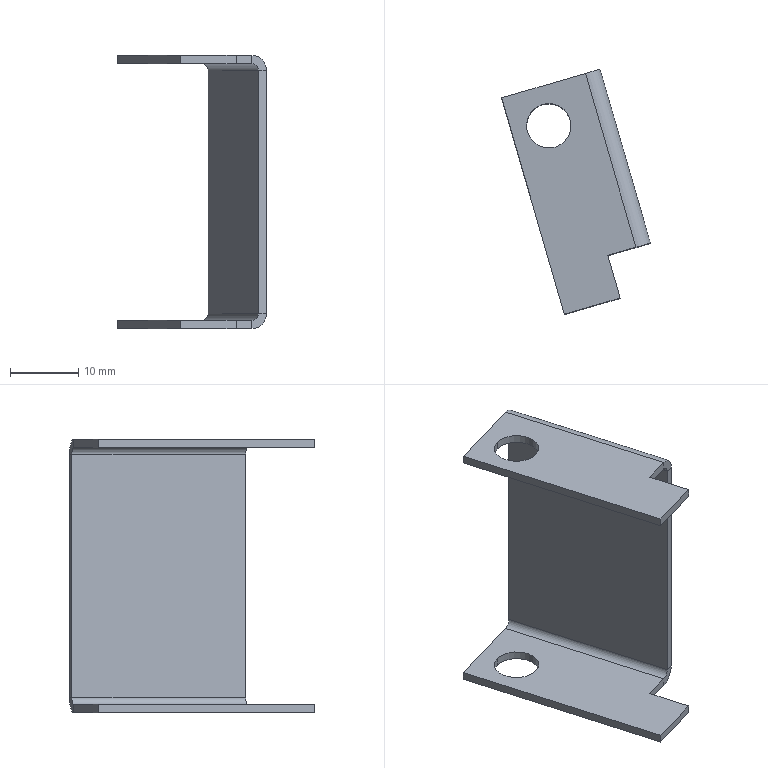Component | SolidWorks | LeftDoorAssembly-1_Bracket-1 | 1 solid | 30 faces | box 21.79 x 35.87 x 40 mm | volume 2159 mm3 | plane 22 | cylinder 8 | commonest cylinder face diameters 6.5 x4 4.4 x2 2 x2
STEP:
#1=CARTESIAN_POINT('',(10.397,8.439,58.906));
#2=VERTEX_POINT('',#1);
#3=CARTESIAN_POINT('',(10.325,8.685,58.906));
#4=VERTEX_POINT('',#3);
#5=CARTESIAN_POINT('',(10.361,8.562,58.906));
#6=DIRECTION('',(-0.,0.,1.));
#7=DIRECTION('',(-0.2786,0.9604,0.));
#8=AXIS2_PLACEMENT_3D('',#5,#6,#7);
#9=CIRCLE('',#8,0.128);
#10=EDGE_CURVE('',#2,#4,#9,.T.);
#11=ORIENTED_EDGE('',*,*,#10,.F.);
#12=CARTESIAN_POINT('',(10.397,8.439,58.953));
#13=VERTEX_POINT('',#12);
#14=CARTESIAN_POINT('',(10.397,8.439,58.906));
#15=DIRECTION('',(-0.,0.,1.));
#16=VECTOR('',#15,39.37);
#17=LINE('',#14,#16);
#18=EDGE_CURVE('',#2,#13,#17,.T.);
#19=ORIENTED_EDGE('',*,*,#18,.T.);
#20=CARTESIAN_POINT('',(10.325,8.685,58.953));
#21=VERTEX_POINT('',#20);
#22=CARTESIAN_POINT('',(10.361,8.562,58.953));
#23=DIRECTION('',(-0.,0.,1.));
#24=DIRECTION('',(-0.2786,0.9604,0.));
#25=AXIS2_PLACEMENT_3D('',#22,#23,#24);
#26=CIRCLE('',#25,0.128);
#27=EDGE_CURVE('',#13,#21,#26,.T.);
#28=ORIENTED_EDGE('',*,*,#27,.T.);
#29=CARTESIAN_POINT('',(10.325,8.685,58.906));
#30=DIRECTION('',(-0.,0.,1.));
#31=VECTOR('',#30,39.37);
#32=LINE('',#29,#31);
#33=EDGE_CURVE('',#4,#21,#32,.T.);
#34=ORIENTED_EDGE('',*,*,#33,.F.);
#35=EDGE_LOOP('',(#11,#19,#28,#34));
#36=FACE_OUTER_BOUND('',#35,.T.);
#37=CARTESIAN_POINT('',(10.361,8.562,58.906));
#38=DIRECTION('',(-0.,0.,1.));
#39=DIRECTION('',(-0.2786,0.9604,0.));
#40=AXIS2_PLACEMENT_3D('',#37,#38,#39);
#41=CYLINDRICAL_SURFACE('',#40,0.128);
#42=ADVANCED_FACE('',(#36),#41,.F.);
#43=CARTESIAN_POINT('',(10.397,8.439,60.433));
#44=VERTEX_POINT('',#43);
#45=CARTESIAN_POINT('',(10.325,8.685,60.433));
#46=VERTEX_POINT('',#45);
#47=CARTESIAN_POINT('',(10.361,8.562,60.433));
#48=DIRECTION('',(-0.,0.,1.));
#49=DIRECTION('',(-0.2786,0.9604,0.));
#50=AXIS2_PLACEMENT_3D('',#47,#48,#49);
#51=CIRCLE('',#50,0.128);
#52=EDGE_CURVE('',#44,#46,#51,.T.);
#53=ORIENTED_EDGE('',*,*,#52,.F.);
#54=CARTESIAN_POINT('',(10.397,8.439,60.48));
#55=VERTEX_POINT('',#54);
#56=CARTESIAN_POINT('',(10.397,8.439,60.48));
#57=DIRECTION('',(-0.,0.,1.));
#58=VECTOR('',#57,39.37);
#59=LINE('',#56,#58);
#60=EDGE_CURVE('',#44,#55,#59,.T.);
#61=ORIENTED_EDGE('',*,*,#60,.T.);
#62=CARTESIAN_POINT('',(10.325,8.685,60.48));
#63=VERTEX_POINT('',#62);
#64=CARTESIAN_POINT('',(10.361,8.562,60.48));
#65=DIRECTION('',(-0.,0.,1.));
#66=DIRECTION('',(-0.2786,0.9604,0.));
#67=AXIS2_PLACEMENT_3D('',#64,#65,#66);
#68=CIRCLE('',#67,0.128);
#69=EDGE_CURVE('',#55,#63,#68,.T.);
#70=ORIENTED_EDGE('',*,*,#69,.T.);
#71=CARTESIAN_POINT('',(10.325,8.685,60.48));
#72=DIRECTION('',(-0.,0.,1.));
#73=VECTOR('',#72,39.37);
#74=LINE('',#71,#73);
#75=EDGE_CURVE('',#46,#63,#74,.T.);
#76=ORIENTED_EDGE('',*,*,#75,.F.);
#77=EDGE_LOOP('',(#53,#61,#70,#76));
#78=FACE_OUTER_BOUND('',#77,.T.);
#79=CARTESIAN_POINT('',(10.361,8.562,60.48));
#80=DIRECTION('',(-0.,0.,1.));
#81=DIRECTION('',(-0.2786,0.9604,0.));
#82=AXIS2_PLACEMENT_3D('',#79,#80,#81);
#83=CYLINDRICAL_SURFACE('',#82,0.128);
#84=ADVANCED_FACE('',(#78),#83,.F.);
#85=CARTESIAN_POINT('',(10.361,8.562,58.906));
#86=DIRECTION('',(-0.,0.,1.));
#87=DIRECTION('',(-0.2786,0.9604,0.));
#88=AXIS2_PLACEMENT_3D('',#85,#86,#87);
#89=CIRCLE('',#88,0.128);
#90=EDGE_CURVE('',#4,#2,#89,.T.);
#91=ORIENTED_EDGE('',*,*,#90,.T.);
#92=ORIENTED_EDGE('',*,*,#10,.T.);
#93=EDGE_LOOP('',(#91,#92));
#94=FACE_BOUND('',#93,.T.);
#95=CARTESIAN_POINT('',(10.863,7.862,58.906));
#96=VERTEX_POINT('',#95);
#97=CARTESIAN_POINT('',(10.573,8.864,58.906));
#98=VERTEX_POINT('',#97);
#99=CARTESIAN_POINT('',(10.935,7.616,58.906));
#100=DIRECTION('',(-0.2786,0.9604,-0.));
#101=VECTOR('',#100,39.37);
#102=LINE('',#99,#101);
#103=EDGE_CURVE('',#96,#98,#102,.T.);
#104=ORIENTED_EDGE('',*,*,#103,.F.);
#105=CARTESIAN_POINT('',(10.701,7.815,58.906));
#106=VERTEX_POINT('',#105);
#107=CARTESIAN_POINT('',(10.901,7.873,58.906));
#108=DIRECTION('',(0.9604,0.2786,0.));
#109=VECTOR('',#108,39.37);
#110=LINE('',#107,#109);
#111=EDGE_CURVE('',#106,#96,#110,.T.);
#112=ORIENTED_EDGE('',*,*,#111,.F.);
#113=CARTESIAN_POINT('',(10.772,7.569,58.906));
#114=VERTEX_POINT('',#113);
#115=CARTESIAN_POINT('',(10.772,7.569,58.906));
#116=DIRECTION('',(-0.2786,0.9604,-0.));
#117=VECTOR('',#116,39.37);
#118=LINE('',#115,#117);
#119=EDGE_CURVE('',#114,#106,#118,.T.);
#120=ORIENTED_EDGE('',*,*,#119,.F.);
#121=CARTESIAN_POINT('',(10.451,7.476,58.906));
#122=VERTEX_POINT('',#121);
#123=CARTESIAN_POINT('',(10.973,7.627,58.906));
#124=DIRECTION('',(-0.9604,-0.2786,-0.));
#125=VECTOR('',#124,39.37);
#126=LINE('',#123,#125);
#127=EDGE_CURVE('',#114,#122,#126,.T.);
#128=ORIENTED_EDGE('',*,*,#127,.T.);
#129=CARTESIAN_POINT('',(10.089,8.723,58.906));
#130=VERTEX_POINT('',#129);
#131=CARTESIAN_POINT('',(10.451,7.476,58.906));
#132=DIRECTION('',(-0.2786,0.9604,-0.));
#133=VECTOR('',#132,39.37);
#134=LINE('',#131,#133);
#135=EDGE_CURVE('',#122,#130,#134,.T.);
#136=ORIENTED_EDGE('',*,*,#135,.T.);
#137=CARTESIAN_POINT('',(10.611,8.875,58.906));
#138=DIRECTION('',(-0.9604,-0.2786,-0.));
#139=VECTOR('',#138,39.37);
#140=LINE('',#137,#139);
#141=EDGE_CURVE('',#98,#130,#140,.T.);
#142=ORIENTED_EDGE('',*,*,#141,.F.);
#143=EDGE_LOOP('',(#104,#112,#120,#128,#136,#142));
#144=FACE_OUTER_BOUND('',#143,.T.);
#145=CARTESIAN_POINT('',(10.973,7.627,58.906));
#146=DIRECTION('',(0.,-0.,-1.));
#147=DIRECTION('',(0.2786,-0.9604,0.));
#148=AXIS2_PLACEMENT_3D('',#145,#146,#147);
#149=PLANE('',#148);
#150=ADVANCED_FACE('',(#94,#144),#149,.T.);
#151=CARTESIAN_POINT('',(10.361,8.562,58.953));
#152=DIRECTION('',(-0.,0.,1.));
#153=DIRECTION('',(-0.2786,0.9604,0.));
#154=AXIS2_PLACEMENT_3D('',#151,#152,#153);
#155=CIRCLE('',#154,0.128);
#156=EDGE_CURVE('',#21,#13,#155,.T.);
#157=ORIENTED_EDGE('',*,*,#156,.F.);
#158=ORIENTED_EDGE('',*,*,#27,.F.);
#159=EDGE_LOOP('',(#157,#158));
#160=FACE_BOUND('',#159,.T.);
#161=CARTESIAN_POINT('',(10.701,7.815,58.953));
#162=VERTEX_POINT('',#161);
#163=CARTESIAN_POINT('',(10.863,7.862,58.953));
#164=VERTEX_POINT('',#163);
#165=CARTESIAN_POINT('',(10.901,7.873,58.953));
#166=DIRECTION('',(0.9604,0.2786,0.));
#167=VECTOR('',#166,39.37);
#168=LINE('',#165,#167);
#169=EDGE_CURVE('',#162,#164,#168,.T.);
#170=ORIENTED_EDGE('',*,*,#169,.T.);
#171=CARTESIAN_POINT('',(10.573,8.864,58.953));
#172=VERTEX_POINT('',#171);
#173=CARTESIAN_POINT('',(10.935,7.616,58.953));
#174=DIRECTION('',(-0.2786,0.9604,-0.));
#175=VECTOR('',#174,39.37);
#176=LINE('',#173,#175);
#177=EDGE_CURVE('',#164,#172,#176,.T.);
#178=ORIENTED_EDGE('',*,*,#177,.T.);
#179=CARTESIAN_POINT('',(10.089,8.723,58.953));
#180=VERTEX_POINT('',#179);
#181=CARTESIAN_POINT('',(10.611,8.875,58.953));
#182=DIRECTION('',(-0.9604,-0.2786,-0.));
#183=VECTOR('',#182,39.37);
#184=LINE('',#181,#183);
#185=EDGE_CURVE('',#172,#180,#184,.T.);
#186=ORIENTED_EDGE('',*,*,#185,.T.);
#187=CARTESIAN_POINT('',(10.451,7.476,58.953));
#188=VERTEX_POINT('',#187);
#189=CARTESIAN_POINT('',(10.451,7.476,58.953));
#190=DIRECTION('',(-0.2786,0.9604,-0.));
#191=VECTOR('',#190,39.37);
#192=LINE('',#189,#191);
#193=EDGE_CURVE('',#188,#180,#192,.T.);
#194=ORIENTED_EDGE('',*,*,#193,.F.);
#195=CARTESIAN_POINT('',(10.772,7.569,58.953));
#196=VERTEX_POINT('',#195);
#197=CARTESIAN_POINT('',(10.973,7.627,58.953));
#198=DIRECTION('',(-0.9604,-0.2786,-0.));
#199=VECTOR('',#198,39.37);
#200=LINE('',#197,#199);
#201=EDGE_CURVE('',#196,#188,#200,.T.);
#202=ORIENTED_EDGE('',*,*,#201,.F.);
#203=CARTESIAN_POINT('',(10.772,7.569,58.953));
#204=DIRECTION('',(-0.2786,0.9604,-0.));
#205=VECTOR('',#204,39.37);
#206=LINE('',#203,#205);
#207=EDGE_CURVE('',#196,#162,#206,.T.);
#208=ORIENTED_EDGE('',*,*,#207,.T.);
#209=EDGE_LOOP('',(#170,#178,#186,#194,#202,#208));
#210=FACE_OUTER_BOUND('',#209,.T.);
#211=CARTESIAN_POINT('',(10.973,7.627,58.953));
#212=DIRECTION('',(0.,-0.,-1.));
#213=DIRECTION('',(0.2786,-0.9604,0.));
#214=AXIS2_PLACEMENT_3D('',#211,#212,#213);
#215=PLANE('',#214);
#216=ADVANCED_FACE('',(#160,#210),#215,.F.);
#217=CARTESIAN_POINT('',(10.361,8.562,60.48));
#218=DIRECTION('',(-0.,0.,1.));
#219=DIRECTION('',(-0.2786,0.9604,0.));
#220=AXIS2_PLACEMENT_3D('',#217,#218,#219);
#221=CIRCLE('',#220,0.128);
#222=EDGE_CURVE('',#63,#55,#221,.T.);
#223=ORIENTED_EDGE('',*,*,#222,.F.);
#224=ORIENTED_EDGE('',*,*,#69,.F.);
#225=EDGE_LOOP('',(#223,#224));
#226=FACE_BOUND('',#225,.T.);
#227=CARTESIAN_POINT('',(10.451,7.476,60.48));
#228=VERTEX_POINT('',#227);
#229=CARTESIAN_POINT('',(10.772,7.569,60.48));
#230=VERTEX_POINT('',#229);
#231=CARTESIAN_POINT('',(10.973,7.627,60.48));
#232=DIRECTION('',(0.9604,0.2786,0.));
#233=VECTOR('',#232,39.37);
#234=LINE('',#231,#233);
#235=EDGE_CURVE('',#228,#230,#234,.T.);
#236=ORIENTED_EDGE('',*,*,#235,.T.);
#237=CARTESIAN_POINT('',(10.701,7.815,60.48));
#238=VERTEX_POINT('',#237);
#239=CARTESIAN_POINT('',(10.772,7.569,60.48));
#240=DIRECTION('',(0.2786,-0.9604,0.));
#241=VECTOR('',#240,39.37);
#242=LINE('',#239,#241);
#243=EDGE_CURVE('',#238,#230,#242,.T.);
#244=ORIENTED_EDGE('',*,*,#243,.F.);
#245=CARTESIAN_POINT('',(10.863,7.862,60.48));
#246=VERTEX_POINT('',#245);
#247=CARTESIAN_POINT('',(10.901,7.873,60.48));
#248=DIRECTION('',(-0.9604,-0.2786,-0.));
#249=VECTOR('',#248,39.37);
#250=LINE('',#247,#249);
#251=EDGE_CURVE('',#246,#238,#250,.T.);
#252=ORIENTED_EDGE('',*,*,#251,.F.);
#253=CARTESIAN_POINT('',(10.573,8.864,60.48));
#254=VERTEX_POINT('',#253);
#255=CARTESIAN_POINT('',(10.935,7.616,60.48));
#256=DIRECTION('',(-0.2786,0.9604,-0.));
#257=VECTOR('',#256,39.37);
#258=LINE('',#255,#257);
#259=EDGE_CURVE('',#246,#254,#258,.T.);
#260=ORIENTED_EDGE('',*,*,#259,.T.);
#261=CARTESIAN_POINT('',(10.089,8.723,60.48));
#262=VERTEX_POINT('',#261);
#263=CARTESIAN_POINT('',(10.611,8.875,60.48));
#264=DIRECTION('',(0.9604,0.2786,0.));
#265=VECTOR('',#264,39.37);
#266=LINE('',#263,#265);
#267=EDGE_CURVE('',#262,#254,#266,.T.);
#268=ORIENTED_EDGE('',*,*,#267,.F.);
#269=CARTESIAN_POINT('',(10.451,7.476,60.48));
#270=DIRECTION('',(-0.2786,0.9604,-0.));
#271=VECTOR('',#270,39.37);
#272=LINE('',#269,#271);
#273=EDGE_CURVE('',#228,#262,#272,.T.);
#274=ORIENTED_EDGE('',*,*,#273,.F.);
#275=EDGE_LOOP('',(#236,#244,#252,#260,#268,#274));
#276=FACE_OUTER_BOUND('',#275,.T.);
#277=CARTESIAN_POINT('',(10.973,7.627,60.48));
#278=DIRECTION('',(-0.,0.,1.));
#279=DIRECTION('',(-0.2786,0.9604,-0.));
#280=AXIS2_PLACEMENT_3D('',#277,#278,#279);
#281=PLANE('',#280);
#282=ADVANCED_FACE('',(#226,#276),#281,.T.);
#283=CARTESIAN_POINT('',(10.361,8.562,60.433));
#284=DIRECTION('',(-0.,0.,1.));
#285=DIRECTION('',(-0.2786,0.9604,0.));
#286=AXIS2_PLACEMENT_3D('',#283,#284,#285);
#287=CIRCLE('',#286,0.128);
#288=EDGE_CURVE('',#46,#44,#287,.T.);
#289=ORIENTED_EDGE('',*,*,#288,.T.);
#290=ORIENTED_EDGE('',*,*,#52,.T.);
#291=EDGE_LOOP('',(#289,#290));
#292=FACE_BOUND('',#291,.T.);
#293=CARTESIAN_POINT('',(10.701,7.815,60.433));
#294=VERTEX_POINT('',#293);
#295=CARTESIAN_POINT('',(10.772,7.569,60.433));
#296=VERTEX_POINT('',#295);
#297=CARTESIAN_POINT('',(10.772,7.569,60.433));
#298=DIRECTION('',(0.2786,-0.9604,0.));
#299=VECTOR('',#298,39.37);
#300=LINE('',#297,#299);
#301=EDGE_CURVE('',#294,#296,#300,.T.);
#302=ORIENTED_EDGE('',*,*,#301,.T.);
#303=CARTESIAN_POINT('',(10.451,7.476,60.433));
#304=VERTEX_POINT('',#303);
#305=CARTESIAN_POINT('',(10.973,7.627,60.433));
#306=DIRECTION('',(0.9604,0.2786,0.));
#307=VECTOR('',#306,39.37);
#308=LINE('',#305,#307);
#309=EDGE_CURVE('',#304,#296,#308,.T.);
#310=ORIENTED_EDGE('',*,*,#309,.F.);
#311=CARTESIAN_POINT('',(10.089,8.723,60.433));
#312=VERTEX_POINT('',#311);
#313=CARTESIAN_POINT('',(10.451,7.476,60.433));
#314=DIRECTION('',(-0.2786,0.9604,-0.));
#315=VECTOR('',#314,39.37);
#316=LINE('',#313,#315);
#317=EDGE_CURVE('',#304,#312,#316,.T.);
#318=ORIENTED_EDGE('',*,*,#317,.T.);
#319=CARTESIAN_POINT('',(10.573,8.864,60.433));
#320=VERTEX_POINT('',#319);
#321=CARTESIAN_POINT('',(10.611,8.875,60.433));
#322=DIRECTION('',(0.9604,0.2786,0.));
#323=VECTOR('',#322,39.37);
#324=LINE('',#321,#323);
#325=EDGE_CURVE('',#312,#320,#324,.T.);
#326=ORIENTED_EDGE('',*,*,#325,.T.);
#327=CARTESIAN_POINT('',(10.863,7.862,60.433));
#328=VERTEX_POINT('',#327);
#329=CARTESIAN_POINT('',(10.935,7.616,60.433));
#330=DIRECTION('',(-0.2786,0.9604,-0.));
#331=VECTOR('',#330,39.37);
#332=LINE('',#329,#331);
#333=EDGE_CURVE('',#328,#320,#332,.T.);
#334=ORIENTED_EDGE('',*,*,#333,.F.);
#335=CARTESIAN_POINT('',(10.901,7.873,60.433));
#336=DIRECTION('',(-0.9604,-0.2786,-0.));
#337=VECTOR('',#336,39.37);
#338=LINE('',#335,#337);
#339=EDGE_CURVE('',#328,#294,#338,.T.);
#340=ORIENTED_EDGE('',*,*,#339,.T.);
#341=EDGE_LOOP('',(#302,#310,#318,#326,#334,#340));
#342=FACE_OUTER_BOUND('',#341,.T.);
#343=CARTESIAN_POINT('',(10.973,7.627,60.433));
#344=DIRECTION('',(-0.,0.,1.));
#345=DIRECTION('',(-0.2786,0.9604,-0.));
#346=AXIS2_PLACEMENT_3D('',#343,#344,#345);
#347=PLANE('',#346);
#348=ADVANCED_FACE('',(#292,#342),#347,.F.);
#349=ORIENTED_EDGE('',*,*,#309,.T.);
#350=CARTESIAN_POINT('',(10.772,7.569,60.433));
#351=DIRECTION('',(-0.,0.,1.));
#352=VECTOR('',#351,39.37);
#353=LINE('',#350,#352);
#354=EDGE_CURVE('',#296,#230,#353,.T.);
#355=ORIENTED_EDGE('',*,*,#354,.T.);
#356=ORIENTED_EDGE('',*,*,#235,.F.);
#357=CARTESIAN_POINT('',(10.451,7.476,60.48));
#358=DIRECTION('',(0.,-0.,-1.));
#359=VECTOR('',#358,39.37);
#360=LINE('',#357,#359);
#361=EDGE_CURVE('',#228,#304,#360,.T.);
#362=ORIENTED_EDGE('',*,*,#361,.T.);
#363=EDGE_LOOP('',(#349,#355,#356,#362));
#364=FACE_OUTER_BOUND('',#363,.T.);
#365=CARTESIAN_POINT('',(11.018,7.64,60.394));
#366=DIRECTION('',(0.2786,-0.9604,0.));
#367=DIRECTION('',(-0.,0.,1.));
#368=AXIS2_PLACEMENT_3D('',#365,#366,#367);
#369=PLANE('',#368);
#370=ADVANCED_FACE('',(#364),#369,.T.);
#371=CARTESIAN_POINT('',(10.947,7.886,58.992));
#372=VERTEX_POINT('',#371);
#373=CARTESIAN_POINT('',(10.656,8.888,58.992));
#374=VERTEX_POINT('',#373);
#375=CARTESIAN_POINT('',(11.018,7.64,58.992));
#376=DIRECTION('',(-0.2786,0.9604,-0.));
#377=VECTOR('',#376,39.37);
#378=LINE('',#375,#377);
#379=EDGE_CURVE('',#372,#374,#378,.T.);
#380=ORIENTED_EDGE('',*,*,#379,.F.);
#381=CARTESIAN_POINT('',(10.863,7.862,58.992));
#382=DIRECTION('',(0.2786,-0.9604,0.));
#383=DIRECTION('',(0.,0.,-1.));
#384=AXIS2_PLACEMENT_3D('',#381,#382,#383);
#385=CIRCLE('',#384,0.08661);
#386=EDGE_CURVE('',#96,#372,#385,.T.);
#387=ORIENTED_EDGE('',*,*,#386,.F.);
#388=ORIENTED_EDGE('',*,*,#103,.T.);
#389=CARTESIAN_POINT('',(10.573,8.864,58.992));
#390=DIRECTION('',(-0.2786,0.9604,-0.));
#391=DIRECTION('',(0.,0.,-1.));
#392=AXIS2_PLACEMENT_3D('',#389,#390,#391);
#393=CIRCLE('',#392,0.08661);
#394=EDGE_CURVE('',#374,#98,#393,.T.);
#395=ORIENTED_EDGE('',*,*,#394,.F.);
#396=EDGE_LOOP('',(#380,#387,#388,#395));
#397=FACE_OUTER_BOUND('',#396,.T.);
#398=CARTESIAN_POINT('',(10.935,7.616,58.992));
#399=DIRECTION('',(-0.2786,0.9604,-0.));
#400=DIRECTION('',(0.,0.,-1.));
#401=AXIS2_PLACEMENT_3D('',#398,#399,#400);
#402=CYLINDRICAL_SURFACE('',#401,0.08661);
#403=ADVANCED_FACE('',(#397),#402,.T.);
#404=CARTESIAN_POINT('',(10.947,7.886,60.394));
#405=VERTEX_POINT('',#404);
#406=CARTESIAN_POINT('',(10.656,8.888,60.394));
#407=VERTEX_POINT('',#406);
#408=CARTESIAN_POINT('',(11.018,7.64,60.394));
#409=DIRECTION('',(-0.2786,0.9604,-0.));
#410=VECTOR('',#409,39.37);
#411=LINE('',#408,#410);
#412=EDGE_CURVE('',#405,#407,#411,.T.);
#413=ORIENTED_EDGE('',*,*,#412,.F.);
#414=CARTESIAN_POINT('',(10.947,7.886,60.433));
#415=DIRECTION('',(-0.,0.,1.));
#416=VECTOR('',#415,39.37);
#417=LINE('',#414,#416);
#418=EDGE_CURVE('',#372,#405,#417,.T.);
#419=ORIENTED_EDGE('',*,*,#418,.F.);
#420=ORIENTED_EDGE('',*,*,#379,.T.);
#421=CARTESIAN_POINT('',(10.656,8.888,60.433));
#422=DIRECTION('',(0.,-0.,-1.));
#423=VECTOR('',#422,39.37);
#424=LINE('',#421,#423);
#425=EDGE_CURVE('',#407,#374,#424,.T.);
#426=ORIENTED_EDGE('',*,*,#425,.F.);
#427=EDGE_LOOP('',(#413,#419,#420,#426));
#428=FACE_OUTER_BOUND('',#427,.T.);
#429=CARTESIAN_POINT('',(11.018,7.64,60.433));
#430=DIRECTION('',(0.9604,0.2786,0.));
#431=DIRECTION('',(0.,-0.,-1.));
#432=AXIS2_PLACEMENT_3D('',#429,#430,#431);
#433=PLANE('',#432);
#434=ADVANCED_FACE('',(#428),#433,.T.);
#435=ORIENTED_EDGE('',*,*,#259,.F.);
#436=CARTESIAN_POINT('',(10.863,7.862,60.394));
#437=DIRECTION('',(0.2786,-0.9604,0.));
#438=DIRECTION('',(0.,0.,-1.));
#439=AXIS2_PLACEMENT_3D('',#436,#437,#438);
#440=CIRCLE('',#439,0.08661);
#441=EDGE_CURVE('',#405,#246,#440,.T.);
#442=ORIENTED_EDGE('',*,*,#441,.F.);
#443=ORIENTED_EDGE('',*,*,#412,.T.);
#444=CARTESIAN_POINT('',(10.573,8.864,60.394));
#445=DIRECTION('',(-0.2786,0.9604,-0.));
#446=DIRECTION('',(0.,0.,-1.));
#447=AXIS2_PLACEMENT_3D('',#444,#445,#446);
#448=CIRCLE('',#447,0.08661);
#449=EDGE_CURVE('',#254,#407,#448,.T.);
#450=ORIENTED_EDGE('',*,*,#449,.F.);
#451=EDGE_LOOP('',(#435,#442,#443,#450));
#452=FACE_OUTER_BOUND('',#451,.T.);
#453=CARTESIAN_POINT('',(10.935,7.616,60.394));
#454=DIRECTION('',(-0.2786,0.9604,-0.));
#455=DIRECTION('',(0.,0.,-1.));
#456=AXIS2_PLACEMENT_3D('',#453,#454,#455);
#457=CYLINDRICAL_SURFACE('',#456,0.08661);
#458=ADVANCED_FACE('',(#452),#457,.T.);
#459=CARTESIAN_POINT('',(10.901,7.873,60.394));
#460=VERTEX_POINT('',#459);
#461=CARTESIAN_POINT('',(10.863,7.862,60.394));
#462=DIRECTION('',(0.2786,-0.9604,0.));
#463=DIRECTION('',(0.,0.,-1.));
#464=AXIS2_PLACEMENT_3D('',#461,#462,#463);
#465=CIRCLE('',#464,0.03937);
#466=EDGE_CURVE('',#460,#328,#465,.T.);
#467=ORIENTED_EDGE('',*,*,#466,.T.);
#468=ORIENTED_EDGE('',*,*,#333,.T.);
#469=CARTESIAN_POINT('',(10.611,8.875,60.394));
#470=VERTEX_POINT('',#469);
#471=CARTESIAN_POINT('',(10.573,8.864,60.394));
#472=DIRECTION('',(-0.2786,0.9604,-0.));
#473=DIRECTION('',(0.,0.,1.));
#474=AXIS2_PLACEMENT_3D('',#471,#472,#473);
#475=CIRCLE('',#474,0.03937);
#476=EDGE_CURVE('',#320,#470,#475,.T.);
#477=ORIENTED_EDGE('',*,*,#476,.T.);
#478=CARTESIAN_POINT('',(10.973,7.627,60.394));
#479=DIRECTION('',(-0.2786,0.9604,-0.));
#480=VECTOR('',#479,39.37);
#481=LINE('',#478,#480);
#482=EDGE_CURVE('',#460,#470,#481,.T.);
#483=ORIENTED_EDGE('',*,*,#482,.F.);
#484=EDGE_LOOP('',(#467,#468,#477,#483));
#485=FACE_OUTER_BOUND('',#484,.T.);
#486=CARTESIAN_POINT('',(10.935,7.616,60.394));
#487=DIRECTION('',(-0.2786,0.9604,-0.));
#488=DIRECTION('',(0.,0.,-1.));
#489=AXIS2_PLACEMENT_3D('',#486,#487,#488);
#490=CYLINDRICAL_SURFACE('',#489,0.03937);
#491=ADVANCED_FACE('',(#485),#490,.F.);
#492=CARTESIAN_POINT('',(10.901,7.873,58.992));
#493=VERTEX_POINT('',#492);
#494=CARTESIAN_POINT('',(10.901,7.873,60.433));
#495=DIRECTION('',(-0.,0.,1.));
#496=VECTOR('',#495,39.37);
#497=LINE('',#494,#496);
#498=EDGE_CURVE('',#493,#460,#497,.T.);
#499=ORIENTED_EDGE('',*,*,#498,.T.);
#500=ORIENTED_EDGE('',*,*,#482,.T.);
#501=CARTESIAN_POINT('',(10.611,8.875,58.992));
#502=VERTEX_POINT('',#501);
#503=CARTESIAN_POINT('',(10.611,8.875,60.433));
#504=DIRECTION('',(0.,-0.,-1.));
#505=VECTOR('',#504,39.37);
#506=LINE('',#503,#505);
#507=EDGE_CURVE('',#470,#502,#506,.T.);
#508=ORIENTED_EDGE('',*,*,#507,.T.);
#509=CARTESIAN_POINT('',(10.973,7.627,58.992));
#510=DIRECTION('',(-0.2786,0.9604,-0.));
#511=VECTOR('',#510,39.37);
#512=LINE('',#509,#511);
#513=EDGE_CURVE('',#493,#502,#512,.T.);
#514=ORIENTED_EDGE('',*,*,#513,.F.);
#515=EDGE_LOOP('',(#499,#500,#508,#514));
#516=FACE_OUTER_BOUND('',#515,.T.);
#517=CARTESIAN_POINT('',(10.973,7.627,60.433));
#518=DIRECTION('',(0.9604,0.2786,0.));
#519=DIRECTION('',(0.,-0.,-1.));
#520=AXIS2_PLACEMENT_3D('',#517,#518,#519);
#521=PLANE('',#520);
#522=ADVANCED_FACE('',(#516),#521,.F.);
#523=CARTESIAN_POINT('',(10.863,7.862,58.992));
#524=DIRECTION('',(0.2786,-0.9604,0.));
#525=DIRECTION('',(0.,0.,-1.));
#526=AXIS2_PLACEMENT_3D('',#523,#524,#525);
#527=CIRCLE('',#526,0.03937);
#528=EDGE_CURVE('',#164,#493,#527,.T.);
#529=ORIENTED_EDGE('',*,*,#528,.T.);
#530=ORIENTED_EDGE('',*,*,#513,.T.);
#531=CARTESIAN_POINT('',(10.573,8.864,58.992));
#532=DIRECTION('',(-0.2786,0.9604,-0.));
#533=DIRECTION('',(0.,0.,1.));
#534=AXIS2_PLACEMENT_3D('',#531,#532,#533);
#535=CIRCLE('',#534,0.03937);
#536=EDGE_CURVE('',#502,#172,#535,.T.);
#537=ORIENTED_EDGE('',*,*,#536,.T.);
#538=ORIENTED_EDGE('',*,*,#177,.F.);
#539=EDGE_LOOP('',(#529,#530,#537,#538));
#540=FACE_OUTER_BOUND('',#539,.T.);
#541=CARTESIAN_POINT('',(10.935,7.616,58.992));
#542=DIRECTION('',(-0.2786,0.9604,-0.));
#543=DIRECTION('',(0.,0.,-1.));
#544=AXIS2_PLACEMENT_3D('',#541,#542,#543);
#545=CYLINDRICAL_SURFACE('',#544,0.03937);
#546=ADVANCED_FACE('',(#540),#545,.F.);
#547=ORIENTED_EDGE('',*,*,#127,.F.);
#548=CARTESIAN_POINT('',(10.772,7.569,58.953));
#549=DIRECTION('',(0.,-0.,-1.));
#550=VECTOR('',#549,39.37);
#551=LINE('',#548,#550);
#552=EDGE_CURVE('',#196,#114,#551,.T.);
#553=ORIENTED_EDGE('',*,*,#552,.F.);
#554=ORIENTED_EDGE('',*,*,#201,.T.);
#555=CARTESIAN_POINT('',(10.451,7.476,58.953));
#556=DIRECTION('',(0.,-0.,-1.));
#557=VECTOR('',#556,39.37);
#558=LINE('',#555,#557);
#559=EDGE_CURVE('',#188,#122,#558,.T.);
#560=ORIENTED_EDGE('',*,*,#559,.T.);
#561=EDGE_LOOP('',(#547,#553,#554,#560));
#562=FACE_OUTER_BOUND('',#561,.T.);
#563=CARTESIAN_POINT('',(10.935,7.616,58.992));
#564=DIRECTION('',(0.2786,-0.9604,0.));
#565=DIRECTION('',(-0.,0.,1.));
#566=AXIS2_PLACEMENT_3D('',#563,#564,#565);
#567=PLANE('',#566);
#568=ADVANCED_FACE('',(#562),#567,.T.);
#569=CARTESIAN_POINT('',(10.611,8.875,60.394));
#570=DIRECTION('',(0.9604,0.2786,0.));
#571=VECTOR('',#570,39.37);
#572=LINE('',#569,#571);
#573=EDGE_CURVE('',#470,#407,#572,.T.);
#574=ORIENTED_EDGE('',*,*,#573,.F.);
#575=ORIENTED_EDGE('',*,*,#476,.F.);
#576=CARTESIAN_POINT('',(10.573,8.864,60.48));
#577=DIRECTION('',(0.,-0.,-1.));
#578=VECTOR('',#577,39.37);
#579=LINE('',#576,#578);
#580=EDGE_CURVE('',#254,#320,#579,.T.);
#581=ORIENTED_EDGE('',*,*,#580,.F.);
#582=ORIENTED_EDGE('',*,*,#449,.T.);
#583=EDGE_LOOP('',(#574,#575,#581,#582));
#584=FACE_OUTER_BOUND('',#583,.T.);
#585=CARTESIAN_POINT('',(10.611,8.875,60.394));
#586=DIRECTION('',(-0.2786,0.9604,-0.));
#587=DIRECTION('',(0.,-0.,-1.));
#588=AXIS2_PLACEMENT_3D('',#585,#586,#587);
#589=PLANE('',#588);
#590=ADVANCED_FACE('',(#584),#589,.T.);
#591=ORIENTED_EDGE('',*,*,#507,.F.);
#592=ORIENTED_EDGE('',*,*,#573,.T.);
#593=ORIENTED_EDGE('',*,*,#425,.T.);
#594=CARTESIAN_POINT('',(10.656,8.888,58.992));
#595=DIRECTION('',(-0.9604,-0.2786,-0.));
#596=VECTOR('',#595,39.37);
#597=LINE('',#594,#596);
#598=EDGE_CURVE('',#374,#502,#597,.T.);
#599=ORIENTED_EDGE('',*,*,#598,.T.);
#600=EDGE_LOOP('',(#591,#592,#593,#599));
#601=FACE_OUTER_BOUND('',#600,.T.);
#602=CARTESIAN_POINT('',(10.573,8.864,60.48));
#603=DIRECTION('',(-0.2786,0.9604,-0.));
#604=DIRECTION('',(0.,-0.,-1.));
#605=AXIS2_PLACEMENT_3D('',#602,#603,#604);
#606=PLANE('',#605);
#607=ADVANCED_FACE('',(#601),#606,.T.);
#608=CARTESIAN_POINT('',(10.573,8.864,58.953));
#609=DIRECTION('',(0.,-0.,-1.));
#610=VECTOR('',#609,39.37);
#611=LINE('',#608,#610);
#612=EDGE_CURVE('',#172,#98,#611,.T.);
#613=ORIENTED_EDGE('',*,*,#612,.F.);
#614=ORIENTED_EDGE('',*,*,#536,.F.);
#615=ORIENTED_EDGE('',*,*,#598,.F.);
#616=ORIENTED_EDGE('',*,*,#394,.T.);
#617=EDGE_LOOP('',(#613,#614,#615,#616));
#618=FACE_OUTER_BOUND('',#617,.T.);
#619=CARTESIAN_POINT('',(10.573,8.864,58.953));
#620=DIRECTION('',(-0.2786,0.9604,-0.));
#621=DIRECTION('',(0.,-0.,-1.));
#622=AXIS2_PLACEMENT_3D('',#619,#620,#621);
#623=PLANE('',#622);
#624=ADVANCED_FACE('',(#618),#623,.T.);
#625=ORIENTED_EDGE('',*,*,#185,.F.);
#626=ORIENTED_EDGE('',*,*,#612,.T.);
#627=ORIENTED_EDGE('',*,*,#141,.T.);
#628=CARTESIAN_POINT('',(10.089,8.723,58.953));
#629=DIRECTION('',(0.,-0.,-1.));
#630=VECTOR('',#629,39.37);
#631=LINE('',#628,#630);
#632=EDGE_CURVE('',#180,#130,#631,.T.);
#633=ORIENTED_EDGE('',*,*,#632,.F.);
#634=EDGE_LOOP('',(#625,#626,#627,#633));
#635=FACE_OUTER_BOUND('',#634,.T.);
#636=CARTESIAN_POINT('',(10.656,8.888,58.992));
#637=DIRECTION('',(-0.2786,0.9604,-0.));
#638=DIRECTION('',(0.,-0.,-1.));
#639=AXIS2_PLACEMENT_3D('',#636,#637,#638);
#640=PLANE('',#639);
#641=ADVANCED_FACE('',(#635),#640,.T.);
#642=CARTESIAN_POINT('',(10.089,8.723,60.48));
#643=DIRECTION('',(0.,-0.,-1.));
#644=VECTOR('',#643,39.37);
#645=LINE('',#642,#644);
#646=EDGE_CURVE('',#262,#312,#645,.T.);
#647=ORIENTED_EDGE('',*,*,#646,.T.);
#648=ORIENTED_EDGE('',*,*,#317,.F.);
#649=ORIENTED_EDGE('',*,*,#361,.F.);
#650=ORIENTED_EDGE('',*,*,#273,.T.);
#651=EDGE_LOOP('',(#647,#648,#649,#650));
#652=FACE_OUTER_BOUND('',#651,.T.);
#653=CARTESIAN_POINT('',(10.451,7.476,60.48));
#654=DIRECTION('',(0.9604,0.2786,0.));
#655=DIRECTION('',(0.,-0.,-1.));
#656=AXIS2_PLACEMENT_3D('',#653,#654,#655);
#657=PLANE('',#656);
#658=ADVANCED_FACE('',(#652),#657,.F.);
#659=ORIENTED_EDGE('',*,*,#632,.T.);
#660=ORIENTED_EDGE('',*,*,#135,.F.);
#661=ORIENTED_EDGE('',*,*,#559,.F.);
#662=ORIENTED_EDGE('',*,*,#193,.T.);
#663=EDGE_LOOP('',(#659,#660,#661,#662));
#664=FACE_OUTER_BOUND('',#663,.T.);
#665=CARTESIAN_POINT('',(10.451,7.476,58.953));
#666=DIRECTION('',(0.9604,0.2786,0.));
#667=DIRECTION('',(0.,-0.,-1.));
#668=AXIS2_PLACEMENT_3D('',#665,#666,#667);
#669=PLANE('',#668);
#670=ADVANCED_FACE('',(#664),#669,.F.);
#671=ORIENTED_EDGE('',*,*,#267,.T.);
#672=ORIENTED_EDGE('',*,*,#580,.T.);
#673=ORIENTED_EDGE('',*,*,#325,.F.);
#674=ORIENTED_EDGE('',*,*,#646,.F.);
#675=EDGE_LOOP('',(#671,#672,#673,#674));
#676=FACE_OUTER_BOUND('',#675,.T.);
#677=CARTESIAN_POINT('',(10.573,8.864,58.992));
#678=DIRECTION('',(0.2786,-0.9604,0.));
#679=DIRECTION('',(-0.,0.,1.));
#680=AXIS2_PLACEMENT_3D('',#677,#678,#679);
#681=PLANE('',#680);
#682=ADVANCED_FACE('',(#676),#681,.F.);
#683=ORIENTED_EDGE('',*,*,#60,.F.);
#684=ORIENTED_EDGE('',*,*,#288,.F.);
#685=ORIENTED_EDGE('',*,*,#75,.T.);
#686=ORIENTED_EDGE('',*,*,#222,.T.);
#687=EDGE_LOOP('',(#683,#684,#685,#686));
#688=FACE_OUTER_BOUND('',#687,.T.);
#689=CARTESIAN_POINT('',(10.361,8.562,60.48));
#690=DIRECTION('',(-0.,0.,1.));
#691=DIRECTION('',(-0.2786,0.9604,0.));
#692=AXIS2_PLACEMENT_3D('',#689,#690,#691);
#693=CYLINDRICAL_SURFACE('',#692,0.128);
#694=ADVANCED_FACE('',(#688),#693,.F.);
#695=ORIENTED_EDGE('',*,*,#18,.F.);
#696=ORIENTED_EDGE('',*,*,#90,.F.);
#697=ORIENTED_EDGE('',*,*,#33,.T.);
#698=ORIENTED_EDGE('',*,*,#156,.T.);
#699=EDGE_LOOP('',(#695,#696,#697,#698));
#700=FACE_OUTER_BOUND('',#699,.T.);
#701=CARTESIAN_POINT('',(10.361,8.562,58.906));
#702=DIRECTION('',(-0.,0.,1.));
#703=DIRECTION('',(-0.2786,0.9604,0.));
#704=AXIS2_PLACEMENT_3D('',#701,#702,#703);
#705=CYLINDRICAL_SURFACE('',#704,0.128);
#706=ADVANCED_FACE('',(#700),#705,.F.);
#707=CARTESIAN_POINT('',(10.863,7.862,58.953));
#708=DIRECTION('',(0.,-0.,-1.));
#709=VECTOR('',#708,39.37);
#710=LINE('',#707,#709);
#711=EDGE_CURVE('',#164,#96,#710,.T.);
#712=ORIENTED_EDGE('',*,*,#711,.F.);
#713=ORIENTED_EDGE('',*,*,#169,.F.);
#714=CARTESIAN_POINT('',(10.701,7.815,58.953));
#715=DIRECTION('',(0.,-0.,-1.));
#716=VECTOR('',#715,39.37);
#717=LINE('',#714,#716);
#718=EDGE_CURVE('',#162,#106,#717,.T.);
#719=ORIENTED_EDGE('',*,*,#718,.T.);
#720=ORIENTED_EDGE('',*,*,#111,.T.);
#721=EDGE_LOOP('',(#712,#713,#719,#720));
#722=FACE_OUTER_BOUND('',#721,.T.);
#723=CARTESIAN_POINT('',(10.901,7.873,58.953));
#724=DIRECTION('',(-0.2786,0.9604,-0.));
#725=DIRECTION('',(0.9604,0.2786,0.));
#726=AXIS2_PLACEMENT_3D('',#723,#724,#725);
#727=PLANE('',#726);
#728=ADVANCED_FACE('',(#722),#727,.F.);
#729=ORIENTED_EDGE('',*,*,#207,.F.);
#730=ORIENTED_EDGE('',*,*,#552,.T.);
#731=ORIENTED_EDGE('',*,*,#119,.T.);
#732=ORIENTED_EDGE('',*,*,#718,.F.);
#733=EDGE_LOOP('',(#729,#730,#731,#732));
#734=FACE_OUTER_BOUND('',#733,.T.);
#735=CARTESIAN_POINT('',(10.772,7.569,58.953));
#736=DIRECTION('',(-0.9604,-0.2786,-0.));
#737=DIRECTION('',(-0.2786,0.9604,-0.));
#738=AXIS2_PLACEMENT_3D('',#735,#736,#737);
#739=PLANE('',#738);
#740=ADVANCED_FACE('',(#734),#739,.F.);
#741=CARTESIAN_POINT('',(10.901,7.873,60.394));
#742=DIRECTION('',(0.9604,0.2786,0.));
#743=VECTOR('',#742,39.37);
#744=LINE('',#741,#743);
#745=EDGE_CURVE('',#460,#405,#744,.T.);
#746=ORIENTED_EDGE('',*,*,#745,.F.);
#747=ORIENTED_EDGE('',*,*,#498,.F.);
#748=CARTESIAN_POINT('',(10.901,7.873,58.992));
#749=DIRECTION('',(0.9604,0.2786,0.));
#750=VECTOR('',#749,39.37);
#751=LINE('',#748,#750);
#752=EDGE_CURVE('',#493,#372,#751,.T.);
#753=ORIENTED_EDGE('',*,*,#752,.T.);
#754=ORIENTED_EDGE('',*,*,#418,.T.);
#755=EDGE_LOOP('',(#746,#747,#753,#754));
#756=FACE_OUTER_BOUND('',#755,.T.);
#757=CARTESIAN_POINT('',(10.901,7.873,60.433));
#758=DIRECTION('',(-0.2786,0.9604,-0.));
#759=DIRECTION('',(-0.,0.,1.));
#760=AXIS2_PLACEMENT_3D('',#757,#758,#759);
#761=PLANE('',#760);
#762=ADVANCED_FACE('',(#756),#761,.F.);
#763=ORIENTED_EDGE('',*,*,#354,.F.);
#764=ORIENTED_EDGE('',*,*,#301,.F.);
#765=CARTESIAN_POINT('',(10.701,7.815,60.433));
#766=DIRECTION('',(-0.,0.,1.));
#767=VECTOR('',#766,39.37);
#768=LINE('',#765,#767);
#769=EDGE_CURVE('',#294,#238,#768,.T.);
#770=ORIENTED_EDGE('',*,*,#769,.T.);
#771=ORIENTED_EDGE('',*,*,#243,.T.);
#772=EDGE_LOOP('',(#763,#764,#770,#771));
#773=FACE_OUTER_BOUND('',#772,.T.);
#774=CARTESIAN_POINT('',(10.772,7.569,60.433));
#775=DIRECTION('',(-0.9604,-0.2786,-0.));
#776=DIRECTION('',(0.2786,-0.9604,0.));
#777=AXIS2_PLACEMENT_3D('',#774,#775,#776);
#778=PLANE('',#777);
#779=ADVANCED_FACE('',(#773),#778,.F.);
#780=ORIENTED_EDGE('',*,*,#769,.F.);
#781=ORIENTED_EDGE('',*,*,#339,.F.);
#782=CARTESIAN_POINT('',(10.863,7.862,60.433));
#783=DIRECTION('',(-0.,0.,1.));
#784=VECTOR('',#783,39.37);
#785=LINE('',#782,#784);
#786=EDGE_CURVE('',#328,#246,#785,.T.);
#787=ORIENTED_EDGE('',*,*,#786,.T.);
#788=ORIENTED_EDGE('',*,*,#251,.T.);
#789=EDGE_LOOP('',(#780,#781,#787,#788));
#790=FACE_OUTER_BOUND('',#789,.T.);
#791=CARTESIAN_POINT('',(10.901,7.873,60.433));
#792=DIRECTION('',(-0.2786,0.9604,-0.));
#793=DIRECTION('',(-0.9604,-0.2786,-0.));
#794=AXIS2_PLACEMENT_3D('',#791,#792,#793);
#795=PLANE('',#794);
#796=ADVANCED_FACE('',(#790),#795,.F.);
#797=ORIENTED_EDGE('',*,*,#786,.F.);
#798=ORIENTED_EDGE('',*,*,#466,.F.);
#799=ORIENTED_EDGE('',*,*,#745,.T.);
#800=ORIENTED_EDGE('',*,*,#441,.T.);
#801=EDGE_LOOP('',(#797,#798,#799,#800));
#802=FACE_OUTER_BOUND('',#801,.T.);
#803=CARTESIAN_POINT('',(10.863,7.862,60.394));
#804=DIRECTION('',(0.2786,-0.9604,0.));
#805=DIRECTION('',(-0.,0.,1.));
#806=AXIS2_PLACEMENT_3D('',#803,#804,#805);
#807=PLANE('',#806);
#808=ADVANCED_FACE('',(#802),#807,.T.);
#809=ORIENTED_EDGE('',*,*,#386,.T.);
#810=ORIENTED_EDGE('',*,*,#752,.F.);
#811=ORIENTED_EDGE('',*,*,#528,.F.);
#812=ORIENTED_EDGE('',*,*,#711,.T.);
#813=EDGE_LOOP('',(#809,#810,#811,#812));
#814=FACE_OUTER_BOUND('',#813,.T.);
#815=CARTESIAN_POINT('',(10.863,7.862,58.992));
#816=DIRECTION('',(0.2786,-0.9604,0.));
#817=DIRECTION('',(-0.,0.,1.));
#818=AXIS2_PLACEMENT_3D('',#815,#816,#817);
#819=PLANE('',#818);
#820=ADVANCED_FACE('',(#814),#819,.T.);
#821=CLOSED_SHELL('',(#42,#84,#150,#216,#282,#348,#370,#403,#434,#458,#491,#522,#546,#568,#590,#607,#624,#641,#658,#670,#682,#694,#706,#728,#740,#762,#779,#796,#808,#820));
#822=MANIFOLD_SOLID_BREP('',#821);
#823=CARTESIAN_POINT('',(0.,0.,0.));
#824=DIRECTION('',(0.,0.,1.));
#825=DIRECTION('',(1.,0.,0.));
#826=AXIS2_PLACEMENT_3D('',#823,#824,#825);
#827=(LENGTH_UNIT()NAMED_UNIT(*)SI_UNIT($,.METRE.));
#828=LENGTH_MEASURE_WITH_UNIT(LENGTH_MEASURE(0.0254),#827);
#829=DIMENSIONAL_EXPONENTS(1.,0.,0.,0.,0.,0.,0.);
#830=(CONVERSION_BASED_UNIT('',#828)LENGTH_UNIT()NAMED_UNIT(#829));
#831=UNCERTAINTY_MEASURE_WITH_UNIT(LENGTH_MEASURE(0.00001),#830,'','');
#832=(NAMED_UNIT(*)PLANE_ANGLE_UNIT()SI_UNIT($,.RADIAN.));
#833=(NAMED_UNIT(*)SI_UNIT($,.STERADIAN.)SOLID_ANGLE_UNIT());
#834=(GEOMETRIC_REPRESENTATION_CONTEXT(3)GLOBAL_UNCERTAINTY_ASSIGNED_CONTEXT((#831))GLOBAL_UNIT_ASSIGNED_CONTEXT((#830,#832,#833))REPRESENTATION_CONTEXT('',''));
#835=ADVANCED_BREP_SHAPE_REPRESENTATION('',(#822,#826),#834);
#836=COLOUR_RGB('',0.7922,0.8196,0.9333);
#837=FILL_AREA_STYLE_COLOUR('',#836);
#838=FILL_AREA_STYLE('',(#837));
#839=SURFACE_STYLE_FILL_AREA(#838);
#840=SURFACE_SIDE_STYLE('',(#839));
#841=SURFACE_STYLE_USAGE(.BOTH.,#840);
#842=PRESENTATION_STYLE_ASSIGNMENT((#841));
#843=STYLED_ITEM('',(#842),#822);
#844=(LENGTH_UNIT()NAMED_UNIT(*)SI_UNIT($,.METRE.));
#845=LENGTH_MEASURE_WITH_UNIT(LENGTH_MEASURE(0.0254),#844);
#846=DIMENSIONAL_EXPONENTS(1.,0.,0.,0.,0.,0.,0.);
#847=(CONVERSION_BASED_UNIT('',#845)LENGTH_UNIT()NAMED_UNIT(#846));
#848=UNCERTAINTY_MEASURE_WITH_UNIT(LENGTH_MEASURE(0.00001),#847,'','');
#849=(NAMED_UNIT(*)PLANE_ANGLE_UNIT()SI_UNIT($,.RADIAN.));
#850=(NAMED_UNIT(*)SI_UNIT($,.STERADIAN.)SOLID_ANGLE_UNIT());
#851=(GEOMETRIC_REPRESENTATION_CONTEXT(3)GLOBAL_UNCERTAINTY_ASSIGNED_CONTEXT((#848))GLOBAL_UNIT_ASSIGNED_CONTEXT((#847,#849,#850))REPRESENTATION_CONTEXT('',''));
#852=MECHANICAL_DESIGN_GEOMETRIC_PRESENTATION_REPRESENTATION('',(#843),#851);
#853=PRESENTATION_LAYER_ASSIGNMENT('','',(#843));